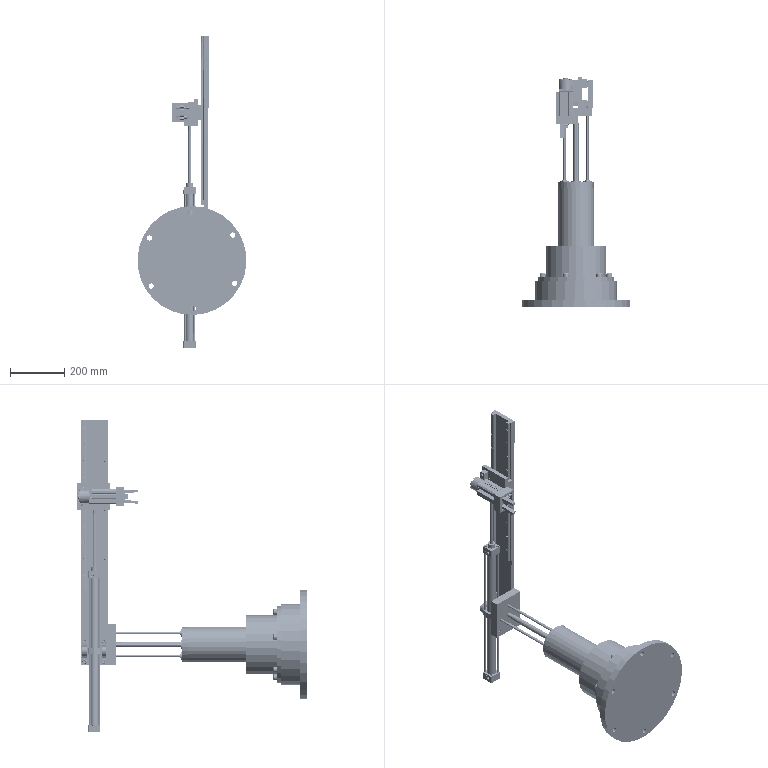Assembly | SolidWorks | mm | 112 component files | 120 solids | 7474 faces | box 400 x 843.52 x 1146.48 mm | volume 16441186 mm3 | plane 3446 | cylinder 1850 | spline 841 | cone 540 | torus 485 | sphere 312 | commonest cylinder face diameters 8 x158 4 x120 14.98 x112 6 x92 15 x81 3 x74 4.8 x68 1 x58
Bill of materials:
15LinearRailSlider | 2 |  | Tall rectangular block with a full-length slot cut into one face; the slot has a profile with small semicircular reliefs at its inner corners. Also has a stepped, counterbored hole on the top face, cross holes on a side face, and a thin raised strip along one side.
15x620LinearRail | 2 |  | Long, slender straight bar with a constant cross-section and a row of evenly spaced small holes along its length. The end profile is roughly I- or hourglass-shaped, with concave cutouts and angled notches on both long sides.
ArmGrippingGear | 2 |  | Straight-toothed spur-gear-like cylinder with a through bore and a single rectangular keyway notch in the bore.
ArmGrippingRack | 1 |  | Rectangular prismatic block with straight, evenly spaced trapezoidal teeth cut along two opposite faces, like a double-sided rack.
ArmRotationCylinderConnectionBlock | 1 |  | Rectangular block with a square cross-section and four round holes in a line along one face: two larger holes near the ends and two smaller holes near the middle.
ArmTelescopicCylinderPistonRod | 1 |  | Long, thin cylindrical rod with a short reduced-diameter step at one end.
Base | 1 |  | Solid round disc with a flange and a raised cylindrical boss on one side. There are six small holes evenly spaced around the edge of the flange.
BearingOuterMountingSleeve | 1 |  | Flanged cylindrical sleeve or tube: a thin annular flange with six small holes evenly spaced around it, joined to a hollow cylindrical body with a large central bore.
ClampingPlate | 2 |  | Rectangular bar with a single round hole near one end, passing across the bar's thickness.
ColumnCylinderPistonRod | 1 |  | Solid cylindrical pin or shaft with one stepped end of reduced diameter.
ColumnLiftingCylinderBody | 1 |  | Multi-body or assembled-looking shape: two square end blocks with rounded corners are joined by a central cylindrical tube and four slender rods, one near each corner. A short cylindrical protrusion sticks out from one end block.
ColumnRotationCylinderFlangePlate | 1 |  | Flat solid disc with a small central bore that has a single rectangular keyway notch.
ColumnSmallArmConnectionPlate | 1 |  | Flat rectangular plate with one larger central hole and eight smaller holes arranged around it: four near the corners and four near the edge midpoints.
CylindricalUpperFlangePlate | 1 |  | Thick round disc with a large central bore and several rings of holes: four large holes, four small inner holes, and four medium holes near the rim.
FixedPost | 1 |  | Straight hollow cylindrical tube with a constant thin wall and plain square-cut ends.
GrippingMandrel | 2 |  | Solid stepped round shaft: a long small-diameter journal at one end, a larger central body with a narrow raised collar, and a short small-diameter stub at the other end.
GrippingMountingHousing | 1 |  | Rectangular block with a large rectangular cavity open on one face. It has a round through-hole centred in the wall opposite the opening and two small holes on an adjacent side face.
GB_FASTENER_SCREWS_HSHCS M3X10-N | 16 |  | Headed cylindrical pin: a short larger-diameter cylindrical head with a rounded outer edge, and a long plain cylindrical shank with a chamfered end.
GB_FASTENER_SCREWS_HSHCS M14X40-N | 6 |  | Headed cylindrical pin with a cylindrical head with a rounded edge and a plain shank with a chamfered tip; the shank is relatively thicker than in similar parts.
GB_FASTENER_SCREWS_HSHCS M6X20-N | 4 |  | Headed cylindrical pin with a cylindrical head with a rounded edge and a long plain chamfered shank.
GB_FASTENER_SCREWS_HSHCS M8X20-N | 4 |  | Headed cylindrical pin with a stubbier shank: a cylindrical head with a rounded edge and a plain chamfered shank.
GB_FASTENER_SCREWS_HSHCS M8X30-N | 4 |  | Slender headed cylindrical pin with a cylindrical head with a rounded edge and a long plain chamfered shank.
GB_FASTENER_SCREWS_HSHCS M10X25-N | 4 |  | Headed cylindrical pin with a relatively large head and a shorter plain chamfered shank.
GB_FASTENER_SCREWS_HSHCS M4X16-N | 28 |  | Long slender headed cylindrical pin with a short cylindrical head with a rounded edge and a long plain chamfered shank.
GB_FASTENER_SCREWS_HSHCS M6X12-N | 2 |  | Stout headed cylindrical pin with a large cylindrical head with a rounded edge and a thick, relatively short plain chamfered shank.
GB_FASTENER_SCREWS_HSHCS M5X20-N | 1 |  | Headed cylindrical part with a hexagonal socket recess in the head; the form resembles a socket-head cap screw, but no threads are modeled.
LiftingRod | 4 |  | Long, slender, solid cylindrical rod with plain ends.
LinearRailConnectionPlate | 1 |  | L-shaped thin plate or bracket: a long narrow upright strip with a short perpendicular return flange at its lower end. Both faces of the lower corner region have a pattern of four small holes.
RackAndPinionRotaryActuatorCDRA1BS50-180CZ | 1 |  | Compact rectangular prismatic body with a square end face. The end face has four socket-head cap screws at its corners. The body has long grooves along its sides, several round side ports or holes, and a cylindrical shaft sticking out from one side face.
MiddleEarFixingBlock1 | 1 |  | Clevis-style bracket: a flat rectangular mounting bar with rounded corners and two through-holes, plus a tapered tongue sticking out perpendicular from the middle of the bar. The tongue ends in a rounded eye with one through-hole.
MiddleEarFixingBlock2 | 1 |  | Clevis-style bracket: a flat rectangular mounting bar with rounded corners and two through-holes, plus a tapered tongue sticking out perpendicular from the middle of the bar. The tongue ends in a rounded eye with one through-hole.
MiddleEarFixingConnectionBlock | 1 |  | Block with a large central through-bore and four smaller through-holes around it. The outline is an irregular hexagon with rectangular tabs on two opposite sides. Two coaxial cylindrical pins (trunnions) stick out from those opposite sides.
RobotArmTelescopicCylinderBody | 1 |  | Long, slender, square-section column: square end caps at both ends, a central tube, and four thin rods running along the corners between the caps. A small round boss with a central hole sticks out from one end cap.
RoundFlangeLinearBearingD8 | 4 |  | Flanged cylindrical bushing or housing: a thin round flange with four equally spaced through-holes and a cylindrical hub on one side. A central through-bore has concentric ring features at the hub end.
SlideRailCarriage | 1 |  | Flat rectangular plate of uniform thickness with ten through-holes: eight small holes in two rectangular four-hole groups and two larger holes arranged vertically near one end.
Rolling bearings 32026 GB 297-94 | 2 |  | Annular rolling-element bearing-like assembly: an outer ring, an inner ring, and a ring of many rolling elements separated by thin webs, with the inner ring standing out axially on one face.
TelescopicCylinderConnectionBlock | 1 |  | Rectangular block with a single round through-hole running through its thickness.
VaneRotaryActuatorCRBU2S30-180 | 1 |  | Housing with a square flange and a cylindrical body. A stepped output shaft with a flat sticks out from the flange face; the body has side pads with holes.
WristClampingCylinderBody | 1 |  | Extruded square-section body with clipped corners, four corner through-holes, a central bore, lengthwise slots or grooves on the outside, and a slotted tab on one side.
WristClampingPistonRod | 1 |  | Stepped round pin or shaft: a long section of larger diameter and a shorter, smaller-diameter section at one end.
Mates:
1. concentric | Base-1 face at (-87.309, 91.019, 566.392) dir (0, -1, 0) r 150 | FixedPost-1 face at (-87.309, 528.019, 566.392) dir (0, -1, 0) r 55
2. concentric | RoundFlangeLinearBearingD8-2 face at (-88.775, 553.019, 608.366) dir (0, 1, 0) r 7.5 | LiftingRod-2 face at (-88.775, 796.583, 608.366) dir (0, -1, 0) r 4
3. width | RackAndPinionRotaryActuatorCDRA1BS50-180CZ-1 face at (-116.161, 145.519, 504.347) dir (-0.9994, 0, -0.0349) | RackAndPinionRotaryActuatorCDRA1BS50-180CZ-1 face at (-54.199, 145.519, 506.511) dir (0.9994, 0, 0.0349) | Base-1 face at (-130.164, 126.019, 647.446) dir (0.9994, 0, 0.0349) | Base-1 face at (-50.213, 126.019, 650.237) dir (-0.9994, 0, -0.0349)
4. width | RackAndPinionRotaryActuatorCDRA1BS50-180CZ-1 face at (-102.231, 186.394, 487.823) dir (0.0349, 0, -0.9994) | RackAndPinionRotaryActuatorCDRA1BS50-180CZ-1 face at (-107.675, 127.644, 643.728) dir (-0.0349, 0, 0.9994) | Base-1 face at (-124.406, 126.019, 482.546) dir (-0.0349, 0, 0.9994) | Base-1 face at (-130.164, 126.019, 647.446) dir (0.0349, 0, -0.9994)
5. coincident | Base-1 face at (-87.309, 126.019, 566.392) dir (0, 1, 0) | RackAndPinionRotaryActuatorCDRA1BS50-180CZ-1 face at (-98.388, 126.019, 504.968) dir (0, -1, 0)
6. concentric | FixedPost-1 face at (-87.309, 528.019, 566.392) dir (0, -1, 0) r 65 | ColumnRotationCylinderFlangePlate-1 face at (-87.309, 208.019, 566.392) dir (0, -1, 0) r 65
7. coincident | RackAndPinionRotaryActuatorCDRA1BS50-180CZ-1 face at (-98.522, 188.019, 543.628) dir (0, 1, 0) | ColumnRotationCylinderFlangePlate-1 face at (-87.309, 188.019, 566.392) dir (0, -1, 0)
8. coincident | FixedPost-1 face at (-87.309, 208.019, 566.392) dir (0, -1, 0) | ColumnRotationCylinderFlangePlate-1 face at (-87.309, 208.019, 566.392) dir (0, 1, 0)
9. concentric | ColumnLiftingCylinderSC50x200-1/ColumnLiftingCylinderBody-1 face at (-87.309, 500.519, 566.392) dir (0, -1, 0) r 25 | FixedPost-1 face at (-87.309, 528.019, 566.392) dir (0, -1, 0) r 65
10. parallel | ColumnLiftingCylinderSC50x200-1/ColumnLiftingCylinderBody-1 face at (-55.354, 235.019, 539.591) dir (0.9994, 0, 0.0349) | Base-1 face at (-130.164, 126.019, 647.446) dir (0.9994, 0, 0.0349)
11. coincident | assembly face at (-87.309, 585.457, 566.392) dir (0, 1, 0) | LiftingRod-2 face at (-88.775, 796.583, 608.366) dir (0, 1, 0)
12. coincident | assembly face at (-87.309, 585.457, 566.392) dir (0, 1, 0) | LiftingRod-2 face at (-88.775, 796.583, 608.366) dir (0, 1, 0)
13. parallel | RobotArmTelescopicCylinderSC32x500-1/MiddleEarFixingBlock1-1 face at (-42.39, 897.583, 491.343) dir (1, 0, -0.00108) | LinearRailConnectionPlate-1 face at (-41.904, 871.583, 941.343) dir (-1, 0, 0.00108)
14. parallel | ColumnSmallArmConnectionPlate-1 face at (-27.228, 806.583, 641.327) dir (1, 0, -0.00108) | LinearRailConnectionPlate-1 face at (-41.904, 871.583, 941.343) dir (-1, 0, 0.00108)
15. coincident | RobotArmTelescopicCylinderSC32x500-1/MiddleEarFixingBlock1-1 face at (-42.39, 897.583, 491.343) dir (1, 0, -0.00108) | LinearRailConnectionPlate-1 face at (-41.904, 871.583, 941.343) dir (-1, 0, 0.00108)
16. width | RobotArmTelescopicCylinderSC32x500-1/MiddleEarFixingBlock2-1 face at (-42.282, 826.583, 591.343) dir (0, -1, 0) | RobotArmTelescopicCylinderSC32x500-1/MiddleEarFixingBlock1-1 face at (-42.282, 916.583, 591.343) dir (0, 1, 0) | LinearRailConnectionPlate-1 face at (-41.418, 921.583, 1391.343) dir (0, 1, 0) | LinearRailConnectionPlate-1 face at (-41.418, 821.583, 1391.343) dir (0, -1, 0)
17. concentric | ColumnLiftingCylinderSC50x200-1/ColumnLiftingCylinderBody-1 face at (-87.309, 527.519, 566.392) dir (0, -1, 0) r 19 | CylindricalUpperFlangePlate-3 face at (-87.309, 548.019, 566.392) dir (0, -1, 0) r 19
18. coincident | ColumnLiftingCylinderSC50x200-1/ColumnLiftingCylinderBody-1 face at (-58.452, 528.019, 539.482) dir (0, 1, 0) | CylindricalUpperFlangePlate-3 face at (-87.309, 528.019, 566.392) dir (0, -1, 0)
19. coincident | FixedPost-1 face at (-87.309, 528.019, 566.392) dir (0, 1, 0) | CylindricalUpperFlangePlate-3 face at (-87.309, 528.019, 566.392) dir (0, -1, 0)
20. parallel | Base-1 face at (-130.164, 126.019, 647.446) dir (0.9994, 0, 0.0349) | CylindricalUpperFlangePlate-3 plane at (-87.309, 528.019, 566.392) dir (0.9994, 0, 0.0349)
21. coincident | RoundFlangeLinearBearingD8-2 face at (-88.775, 553.019, 608.366) dir (0, 1, 0) r 7.5 | CylindricalUpperFlangePlate-3 edge at (-88.775, 548.019, 608.366) dir (0, 1, 0) r 7.5
22. coincident | RoundFlangeLinearBearingD8-2 face at (-88.377, 548.019, 592.371) dir (0, -1, 0) | CylindricalUpperFlangePlate-3 face at (-87.309, 548.019, 566.392) dir (0, 1, 0)
23. width | LinearRailConnectionPlate-1 face at (-42.39, 921.583, 491.343) dir (-0.00108, 0, -1) | LinearRailConnectionPlate-1 face at (-27.228, 821.583, 641.327) dir (0.00108, 0, 1) | ColumnSmallArmConnectionPlate-1 face at (-27.228, 806.583, 641.327) dir (0.00108, 0, 1) | ColumnSmallArmConnectionPlate-1 face at (-27.39, 806.583, 491.327) dir (-0.00108, 0, -1)
24. concentric | assembly face at (-87.309, 585.457, 566.392) dir (0, -1, 0) r 8 | ColumnSmallArmConnectionPlate-1 sketch segment at (-87.309, 806.583, 566.392) dir (0, 1, 0) r 19
25. coincident | ColumnSmallArmConnectionPlate-1 face at (-27.228, 806.583, 641.327) dir (1, 0, -0.00108) | LinearRailConnectionPlate-1 face at (-26.904, 871.583, 941.327) dir (1, 0, -0.00108)
26. coincident | ColumnSmallArmConnectionPlate-1 face at (-87.309, 806.583, 566.392) dir (0, 1, 0) | LinearRailConnectionPlate-1 face at (-27.39, 806.583, 491.327) dir (0, -1, 0)
27. parallel | Base-1 face at (-50.213, 126.019, 650.237) dir (-0.9994, 0, -0.0349) | CylindricalUpperFlangePlate-3 plane at (-87.309, 528.019, 566.392) dir (0.9994, 0, 0.0349)
28. concentric | RoundFlangeLinearBearingD8-2 edge at (-100.771, 549.719, 608.068) dir (0, -1, 0) r 1.7 | CylindricalUpperFlangePlate-3 edge at (-100.771, 548.019, 608.068) dir (0, 1, 0) r 1.5
29. concentric | RoundFlangeLinearBearingD8-2 face at (-89.073, 548.019, 620.362) dir (0, -1, 0) r 3.25 | hexagon socket head cap screws gb-1 face at (-89.073, 539.719, 620.362) dir (0, 1, 0) r 1.5
30. coincident | RoundFlangeLinearBearingD8-2 face at (-89.154, 549.719, 623.611) dir (0, 1, 0) | hexagon socket head cap screws gb-1 face at (-89.073, 549.719, 620.362) dir (0, -1, 0)
31. concentric | CylindricalUpperFlangePlate-3 edge at (-109.975, 541.219, 542.086) dir (0, 1, 0) r 3.3 | hexagon socket head cap screws gb-17 edge at (-109.975, 541.219, 542.086) dir (0, -1, 0) r 3
32. coincident | CylindricalUpperFlangePlate-3 face at (-106.677, 541.219, 542.201) dir (0, 1, 0) | hexagon socket head cap screws gb-17 face at (-109.975, 541.219, 542.086) dir (0, -1, 0)
33. concentric | LinearRailConnectionPlate-1 face at (-132.363, 821.583, 516.44) dir (0, 1, 0) r 7.5 | hexagon socket head cap screws gb-21 face at (-132.363, 792.583, 516.44) dir (0, 1, 0) r 4
34. coincident | LinearRailConnectionPlate-1 face at (-136.863, 812.583, 516.445) dir (0, 1, 0) | hexagon socket head cap screws gb-21 face at (-132.363, 812.583, 516.44) dir (0, -1, 0)
35. concentric | CylindricalUpperFlangePlate-3 face at (-131.19, 548.019, 607.312) dir (0, 1, 0) r 4.25 | hexagon socket head cap screws gb-25 face at (-131.19, 518.019, 607.312) dir (0, 1, 0) r 4
36. coincident | CylindricalUpperFlangePlate-3 face at (-87.309, 548.019, 566.392) dir (0, 1, 0) | hexagon socket head cap screws gb-25 face at (-131.19, 548.019, 607.312) dir (0, -1, 0)
37. concentric | FixedPost-1 face at (-87.309, 528.019, 566.392) dir (0, -1, 0) r 65 | tapered roller bearings gb-10 face at (-87.309, 306.019, 566.392) dir (0, 1, 0) r 65
38. concentric | FixedPost-1 face at (-87.309, 528.019, 566.392) dir (0, -1, 0) r 65 | tapered roller bearings gb-9 face at (-87.309, 208.019, 566.392) dir (0, -1, 0) r 65
39. concentric | Base-1 face at (-87.309, 91.019, 566.392) dir (0, -1, 0) r 150 | BearingOuterMountingSleeve-1 face at (-87.309, 186.019, 566.392) dir (0, -1, 0) r 110
40. coincident | Base-1 face at (-87.309, 186.019, 566.392) dir (0, 1, 0) | BearingOuterMountingSleeve-1 face at (-21.667, 186.019, 641.832) dir (0, -1, 0)
41. coincident | FixedPost-1 edge at (-87.309, 208.019, 566.392) dir (0, 1, 0) r 65 | tapered roller bearings gb-9 face at (-87.309, 208.019, 566.392) dir (0, -1, 0)
42. coincident | tapered roller bearings gb-10 face at (-87.309, 306.019, 566.392) dir (0, 1, 0) | BearingOuterMountingSleeve-1 edge at (-87.309, 306.019, 566.392) dir (0, 1, 0) r 65
43. concentric | ColumnSmallArmConnectionPlate-1 face at (-85.843, 791.583, 524.417) dir (0, -1, 0) r 4 | LiftingRod-4 face at (-85.843, 796.583, 524.417) dir (0, -1, 0) r 4
44. concentric | ColumnSmallArmConnectionPlate-1 face at (-129.284, 791.583, 564.926) dir (0, -1, 0) r 4 | LiftingRod-3 face at (-129.284, 796.583, 564.926) dir (0, -1, 0) r 4
45. concentric | ColumnSmallArmConnectionPlate-1 face at (-88.775, 791.583, 608.366) dir (0, -1, 0) r 4 | LiftingRod-2 face at (-88.775, 796.583, 608.366) dir (0, -1, 0) r 4
46. coincident | RobotArmTelescopicCylinderSC32x500-1/MiddleEarFixingBlock1-1 face at (-53.39, 897.583, 491.355) dir (-0.00108, 0, -1) | LinearRailConnectionPlate-1 face at (-42.39, 921.583, 491.343) dir (-0.00108, 0, -1)
47. coincident | LinearRailConnectionPlate-1 face at (-41.904, 871.583, 941.343) dir (-1, 0, 0.00108) | 15x620LinearRail-1 face at (-41.418, 904.112, 1391.343) dir (1, 0, -0.00108)
48. parallel | LinearRailConnectionPlate-1 face at (-41.418, 921.583, 1391.343) dir (0, 1, 0) | 15x620LinearRail-1 face at (-48.317, 916.583, 1391.35) dir (0, 1, 0)
49. coincident | LinearRailConnectionPlate-1 face at (-41.418, 921.583, 1391.343) dir (0.00108, 0, 1) | 15x620LinearRail-1 face at (-43.31, 918.112, 1391.345) dir (0.00108, 0, 1)
50. distance | 15x620LinearRail-1 face at (-48.317, 916.583, 1391.35) dir (0, 1, 0) | LinearRailConnectionPlate-1 face at (-41.418, 921.583, 1391.343) dir (0, 1, 0)
51. width | 15LinearRailSlider-1 face at (-46.073, 916.792, 1081.267) dir (0, -1, 0) | 15LinearRailSlider-1 face at (-48.605, 905.432, 1081.27) dir (0, 1, 0) | 15x620LinearRail-1 face at (-52.248, 918.612, 1391.354) dir (0, 1, 0) | 15x620LinearRail-1 face at (-52.248, 903.612, 1391.354) dir (0, -1, 0)
52. coincident | 15x620LinearRail-1 face at (-53.918, 916.942, 1391.356) dir (-1, 0, 0.00108) | 15LinearRailSlider-1 face at (-54.253, 916.942, 1081.276) dir (1, 0, -0.00108)
53. concentric | RobotArmTelescopicCylinderSC32x500-1/MiddleEarFixingBlock1-1 edge at (-53.377, 907.083, 503.855) dir (1, 0, -0.00108) r 6 | hexagon socket head cap screws gb-29 edge at (-53.377, 907.083, 503.855) dir (1, 0, -0.00108) r 5
54. coincident | RobotArmTelescopicCylinderSC32x500-1/MiddleEarFixingBlock1-1 face at (-53.282, 897.583, 591.355) dir (-1, 0, 0.00108) | hexagon socket head cap screws gb-29 face at (-53.377, 907.083, 503.855) dir (1, 0, -0.00108)
55. concentric | 15x620LinearRail-1 face at (-54.534, 911.112, 821.356) dir (-1, 0, 0.00108) r 4 | hexagon socket head cap screws gb-34 face at (-33.934, 911.112, 821.334) dir (-1, 0, 0.00108) r 2
56. coincident | 15x620LinearRail-1 face at (-49.934, 913.512, 821.352) dir (-1, 0, 0.00108) | hexagon socket head cap screws gb-34 face at (-49.934, 911.112, 821.352) dir (1, 0, -0.00108)
57. concentric | 15x620LinearRail-3 face at (-53.95, 832.054, 1361.356) dir (-1, 0, 0.00108) r 4 | hexagon socket head cap screws gb-64 face at (-33.35, 832.054, 1361.334) dir (-1, 0, 0.00108) r 2
58. coincident | 15x620LinearRail-3 edge at (-49.35, 832.054, 1361.351) dir (-1, 0, 0.00108) r 4 | hexagon socket head cap screws gb-64 face at (-49.35, 832.054, 1361.351) dir (1, 0, -0.00108)
59. coincident | SlideRailCarriage-1 face at (-65.542, 874.54, 1109.688) dir (1, 0, -0.00108) | 15LinearRailSlider-1 face at (-65.395, 866.112, 1245.688) dir (-1, 0, 0.00108)
60. width | SlideRailCarriage-1 face at (-65.488, 934.54, 1159.688) dir (0.00108, 0, 1) | SlideRailCarriage-1 face at (-65.596, 934.54, 1059.688) dir (-0.00108, 0, -1) | 15LinearRailSlider-1 face at (-43.512, 866.112, 1138.065) dir (0.00108, 0, 1) | 15LinearRailSlider-1 face at (-43.573, 866.112, 1081.265) dir (-0.00108, 0, -1)
61. coincident | SlideRailCarriage-1 face at (-80.542, 874.54, 1109.705) dir (-1, 0, 0.00108) | ArmRotationCylinderConnectionBlock-1 face at (-80.499, 924.54, 1149.704) dir (1, 0, -0.00108)
62. concentric | SlideRailCarriage-1 face at (-80.556, 845.054, 1096.705) dir (-1, 0, 0.00108) r 2.25 | hexagon socket head cap screws gb-75 face at (-59.956, 845.054, 1096.682) dir (-1, 0, 0.00108) r 2
63. coincident | SlideRailCarriage-1 face at (-75.956, 842.804, 1096.7) dir (-1, 0, 0.00108) | hexagon socket head cap screws gb-75 face at (-75.956, 845.054, 1096.7) dir (1, 0, -0.00108)
64. concentric | SlideRailCarriage-1 face at (-80.528, 845.054, 1122.705) dir (-1, 0, 0.00108) r 2.25 | hexagon socket head cap screws gb-76 face at (-59.928, 845.054, 1122.682) dir (-1, 0, 0.00108) r 2
65. coincident | SlideRailCarriage-1 face at (-75.928, 842.804, 1122.7) dir (-1, 0, 0.00108) | hexagon socket head cap screws gb-76 face at (-75.928, 845.054, 1122.7) dir (1, 0, -0.00108)
66. concentric | SlideRailCarriage-1 face at (-80.556, 819.054, 1096.705) dir (-1, 0, 0.00108) r 2.25 | hexagon socket head cap screws gb-77 face at (-59.956, 819.054, 1096.682) dir (-1, 0, 0.00108) r 2
67. coincident | SlideRailCarriage-1 face at (-75.956, 816.804, 1096.7) dir (-1, 0, 0.00108) | hexagon socket head cap screws gb-77 face at (-75.956, 819.054, 1096.7) dir (1, 0, -0.00108)
68. concentric | SlideRailCarriage-1 face at (-80.528, 819.054, 1122.705) dir (-1, 0, 0.00108) r 2.25 | hexagon socket head cap screws gb-78 face at (-59.928, 819.054, 1122.682) dir (-1, 0, 0.00108) r 2
69. coincident | SlideRailCarriage-1 face at (-75.928, 816.804, 1122.7) dir (-1, 0, 0.00108) | hexagon socket head cap screws gb-78 face at (-75.928, 819.054, 1122.7) dir (1, 0, -0.00108)
70. concentric | SlideRailCarriage-1 face at (-80.528, 924.112, 1122.705) dir (-1, 0, 0.00108) r 2.25 | hexagon socket head cap screws gb-79 face at (-59.928, 924.112, 1122.682) dir (-1, 0, 0.00108) r 2
71. coincident | SlideRailCarriage-1 face at (-75.928, 921.862, 1122.7) dir (-1, 0, 0.00108) | hexagon socket head cap screws gb-79 face at (-75.928, 924.112, 1122.7) dir (1, 0, -0.00108)
72. concentric | SlideRailCarriage-1 face at (-80.556, 924.112, 1096.705) dir (-1, 0, 0.00108) r 2.25 | hexagon socket head cap screws gb-80 face at (-59.956, 924.112, 1096.682) dir (-1, 0, 0.00108) r 2
73. coincident | SlideRailCarriage-1 face at (-75.956, 921.862, 1096.7) dir (-1, 0, 0.00108) | hexagon socket head cap screws gb-80 face at (-75.956, 924.112, 1096.7) dir (1, 0, -0.00108)
74. concentric | SlideRailCarriage-1 face at (-80.556, 898.112, 1096.705) dir (-1, 0, 0.00108) r 2.25 | hexagon socket head cap screws gb-81 face at (-59.956, 898.112, 1096.682) dir (-1, 0, 0.00108) r 2
75. coincident | SlideRailCarriage-1 face at (-75.956, 895.862, 1096.7) dir (-1, 0, 0.00108) | hexagon socket head cap screws gb-81 face at (-75.956, 898.112, 1096.7) dir (1, 0, -0.00108)
76. concentric | SlideRailCarriage-1 face at (-80.528, 898.112, 1122.705) dir (-1, 0, 0.00108) r 2.25 | hexagon socket head cap screws gb-82 face at (-59.928, 898.112, 1122.682) dir (-1, 0, 0.00108) r 2
77. coincident | SlideRailCarriage-1 face at (-75.928, 895.862, 1122.7) dir (-1, 0, 0.00108) | hexagon socket head cap screws gb-82 face at (-75.928, 898.112, 1122.7) dir (1, 0, -0.00108)
78. width | ArmRotationCylinderConnectionBlock-1 face at (-100.499, 924.54, 1149.726) dir (0.00108, 0, 1) | ArmRotationCylinderConnectionBlock-1 face at (-100.585, 924.54, 1069.726) dir (-0.00108, 0, -1) | SlideRailCarriage-1 face at (-65.596, 934.54, 1059.688) dir (-0.00108, 0, -1) | SlideRailCarriage-1 face at (-65.488, 934.54, 1159.688) dir (0.00108, 0, 1)
79. concentric | SlideRailCarriage-1 face at (-80.575, 914.54, 1079.705) dir (-1, 0, 0.00108) r 3 | ArmRotationCylinderConnectionBlock-1 face at (-100.575, 914.54, 1079.726) dir (-1, 0, 0.00108) r 5.5
80. concentric | VaneRotaryActuatorCRBU2S30-180-1 face at (-110.05, 914.54, 1102.736) dir (1, 0, -0.00108) r 2.5 | ArmRotationCylinderConnectionBlock-1 edge at (-100.55, 914.54, 1102.726) dir (1, 0, -0.00108) r 2.75
81. coincident | VaneRotaryActuatorCRBU2S30-180-1 face at (-100.555, 902.54, 1097.726) dir (1, 0, -0.00108) | ArmRotationCylinderConnectionBlock-1 face at (-100.499, 924.54, 1149.726) dir (-1, 0, 0.00108)
82. concentric | ArmRotationCylinderConnectionBlock-1 face at (-100.51, 914.54, 1139.726) dir (-1, 0, 0.00108) r 3.3 | hexagon socket head cap screws gb-88 face at (-74.51, 914.54, 1139.698) dir (-1, 0, 0.00108) r 3
83. coincident | ArmRotationCylinderConnectionBlock-1 face at (-86.51, 917.84, 1139.711) dir (-1, 0, 0.00108) | hexagon socket head cap screws gb-88 face at (-86.51, 914.54, 1139.711) dir (1, 0, -0.00108)
84. concentric | ArmRotationCylinderConnectionBlock-1 face at (-100.575, 914.54, 1079.726) dir (-1, 0, 0.00108) r 3.3 | hexagon socket head cap screws gb-89 face at (-74.575, 914.54, 1079.698) dir (-1, 0, 0.00108) r 3
85. coincident | ArmRotationCylinderConnectionBlock-1 face at (-86.575, 917.84, 1079.711) dir (-1, 0, 0.00108) | hexagon socket head cap screws gb-89 face at (-86.575, 914.54, 1079.711) dir (1, 0, -0.00108)
86. concentric | ArmRotationCylinderConnectionBlock-1 face at (-80.535, 914.54, 1116.705) dir (1, 0, -0.00108) r 2.75 | hexagon socket head cap screws gb-94 face at (-106.235, 914.54, 1116.732) dir (1, 0, -0.00108) r 2.5
87. coincident | ArmRotationCylinderConnectionBlock-1 face at (-86.235, 917.29, 1116.711) dir (1, 0, -0.00108) | hexagon socket head cap screws gb-94 face at (-86.235, 914.54, 1116.711) dir (-1, 0, 0.00108)
88. coincident | SlideRailCarriage-1 face at (-80.542, 874.54, 1109.705) dir (-1, 0, 0.00108) | TelescopicCylinderConnectionBlock-1 face at (-80.58, 904.54, 1074.705) dir (1, 0, -0.00108)
89. coincident | ArmRotationCylinderConnectionBlock-1 face at (-90.542, 904.54, 1109.715) dir (0, -1, 0) | TelescopicCylinderConnectionBlock-1 face at (-98.088, 904.54, 1067.223) dir (0, 1, 0)
90. coincident | SlideRailCarriage-1 face at (-65.596, 934.54, 1059.688) dir (-0.00108, 0, -1) | TelescopicCylinderConnectionBlock-1 face at (-115.596, 904.54, 1059.742) dir (-0.00108, 0, -1)
91. concentric | RobotArmTelescopicCylinderSC32x500-1/RobotArmTelescopicCylinderBody-1 face at (-96.627, 871.583, 272.402) dir (0.00108, 0, 1) r 6 | ArmTelescopicCylinderPistonRod-1 face at (-95.792, 871.583, 1044.721) dir (-0.00108, 0, -1) r 6
92. distance | ArmTelescopicCylinderPistonRod-1 face at (-95.771, 871.583, 1064.721) dir (0.00108, 0, 1) | TelescopicCylinderConnectionBlock-1 face at (-115.58, 904.54, 1074.742) dir (0.00108, 0, 1)
93. concentric | CylindricalUpperFlangePlate-3 face at (-87.309, 548.019, 566.392) dir (0, -1, 0) r 19 | ColumnCylinderPistonRod-1 face at (-87.309, 766.583, 566.392) dir (0, -1, 0) r 10
94. coincident | LiftingRod-3 face at (-129.284, 796.583, 564.926) dir (0, 1, 0) | ColumnCylinderPistonRod-1 face at (-87.309, 796.583, 566.392) dir (0, 1, 0)
95. distance | ColumnCylinderPistonRod-1 face at (-87.309, 796.583, 566.392) dir (0, 1, 0) | LinearRailConnectionPlate-1 face at (-27.39, 821.583, 491.327) dir (0, 1, 0)
96. coincident | WristClampingAirCTACQS40x50-1/WristClampingCylinderBody-1 face at (-146.265, 881.04, 1088.576) dir (0, 1, 0) | VaneRotaryActuatorCRBU2S30-180-1 face at (-125.542, 881.04, 1109.753) dir (0, -1, 0)
97. parallel | WristClampingAirCTACQS40x50-1/WristClampingCylinderBody-1 face at (-162.049, 899.632, 1103.469) dir (-1, 0, 0.00108) | SlideRailCarriage-1 face at (-80.542, 874.54, 1109.705) dir (-1, 0, 0.00108)
98. concentric | VaneRotaryActuatorCRBU2S30-180-1 face at (-110.035, 914.54, 1116.736) dir (1, 0, -0.00108) r 2.5 | hexagon socket head cap screws gb-94 face at (-106.235, 914.54, 1116.732) dir (1, 0, -0.00108) r 2.5
99. width | WristClampingAirCTACQS40x50-1/WristClampingCylinderBody-1 face at (-146.271, 881.04, 1083.276) dir (-0.00108, 0, -1) | WristClampingAirCTACQS40x50-1/WristClampingCylinderBody-1 face at (-146.213, 881.04, 1136.275) dir (0.00108, 0, 1) | VaneRotaryActuatorCRBU2S30-180-1 face at (-115.895, 890.04, 1135.743) dir (0.00108, 0, 1) | VaneRotaryActuatorCRBU2S30-180-1 face at (-135.189, 890.04, 1083.764) dir (-0.00108, 0, -1)
100. coincident | WristClampingAirCTACQS40x50-1/WristClampingCylinderBody-1 face at (-151.519, 881.04, 1130.981) dir (-1, 0, 0.00108) | VaneRotaryActuatorCRBU2S30-180-1 face at (-151.553, 890.04, 1100.162) dir (-1, 0, 0.00108)
101. concentric | WristClampingAirCTACQS40x50-1/WristClampingCylinderBody-1 face at (-125.042, 874.04, 1109.753) dir (0, -1, 0) r 8 | WristClampingPistonRod-2 face at (-125.042, 776.966, 1109.753) dir (0, 1, 0) r 6
102. concentric | TelescopicCylinderConnectionBlock-1 face at (-95.76, 871.583, 1074.721) dir (0.00108, 0, 1) r 5 | ArmTelescopicCylinderPistonRod-1 face at (-95.771, 871.583, 1064.721) dir (-0.00108, 0, -1) r 5
103. parallel | SlideRailCarriage-1 face at (-80.542, 874.54, 1109.705) dir (-1, 0, 0.00108) | ArmGrippingRack-1 face at (-132.552, 775.395, 1100.736) dir (-1, 0, 0.00108)
104. parallel | SlideRailCarriage-1 face at (-80.542, 874.54, 1109.705) dir (-1, 0, 0.00108) | ArmGrippingGear-1 face at (-117.551, 768.611, 1101.127) dir (1, 0, -0.00108)
105. concentric | WristClampingPistonRod-2 face at (-125.042, 756.966, 1109.753) dir (0, 1, 0) r 4 | ArmGrippingRack-1 face at (-125.042, 756.966, 1109.753) dir (0, 1, 0) r 5
106. coincident | WristClampingPistonRod-2 face at (-125.042, 776.966, 1109.753) dir (0, -1, 0) | ArmGrippingRack-1 face at (-117.531, 776.966, 1119.769) dir (0, 1, 0)
107. rack pinion | ArmGrippingRack-1 sketch segment at (-125.052, 775.395, 1100.728) dir (0, -1, 0) | ArmGrippingGear-1 sketch segment at (-125.061, 765.309, 1092.228) dir (-1, 0, 0.00108) r 8.5
108. coincident | ArmGrippingRack-1 face at (-132.552, 775.395, 1100.736) dir (-1, 0, 0.00108) | ArmGrippingGear-1 face at (-132.561, 765.309, 1092.236) dir (-1, 0, 0.00108)
109. distance | ArmGrippingGear-1 sketch point at (-125.061, 765.309, 1092.228) dir (1, 0, 0) | ArmGrippingRack-1 sketch segment at (-125.052, 775.395, 1100.728) dir (0, -1, 0)
110. concentric | ArmGrippingGear-1 face at (-125.061, 765.309, 1092.228) dir (-1, 0, 0.00108) r 5 | GrippingMandrel-1 face at (-114.642, 765.309, 1092.216) dir (1, 0, -0.00108) r 5
111. concentric | GrippingMandrel-1 face at (-147.642, 765.309, 1092.252) dir (1, 0, -0.00108) r 3 | ClampingPlate-1 face at (-127.642, 765.309, 1092.23) dir (-1, 0, 0.00108) r 3
112. lock | ArmGrippingGear-1 reference at (0, 0, 0) dir (1, 0, 0) | ClampingPlate-1 reference at (0, 0, 0) dir (1, 0, 0)
113. lock | ArmGrippingGear-2 reference at (0, 0, 0) dir (1, 0, 0) | ClampingPlate-3 reference at (0, 0, 0) dir (1, 0, 0)
114. coincident | GrippingMandrel-1 face at (-147.642, 765.309, 1092.252) dir (-1, 0, 0.00108) | ClampingPlate-1 face at (-147.643, 740.362, 1090.631) dir (-1, 0, 0.00108)
115. coincident | GrippingMandrel-1 face at (-147.642, 765.309, 1092.252) dir (-1, 0, 0.00108) | ClampingPlate-1 face at (-147.643, 740.362, 1090.631) dir (-1, 0, 0.00108)
116. coincident | WristClampingAirCTACQS40x50-1/WristClampingCylinderBody-1 face at (-146.265, 791.54, 1088.576) dir (0, -1, 0) | GrippingMountingHousing-2 face at (-92.004, 791.54, 1144.717) dir (0, 1, 0)
117. width | GrippingMountingHousing-2 face at (-92.004, 791.54, 1144.717) dir (0.00108, 0, 1) | GrippingMountingHousing-2 face at (-92.08, 791.54, 1074.717) dir (-0.00108, 0, -1) | WristClampingAirCTACQS40x50-1/WristClampingCylinderBody-1 face at (-146.271, 881.04, 1083.276) dir (-0.00108, 0, -1) | WristClampingAirCTACQS40x50-1/WristClampingCylinderBody-1 face at (-146.213, 881.04, 1136.275) dir (0.00108, 0, 1)
118. coincident | WristClampingAirCTACQS40x50-1/WristClampingCylinderBody-1 face at (-162.049, 899.632, 1103.469) dir (-1, 0, 0.00108) | GrippingMountingHousing-2 face at (-162.042, 776.54, 1109.793) dir (-1, 0, 0.00108)
119. concentric | BearingOuterMountingSleeve-1 face at (-209.195, 201.019, 594.437) dir (0, 1, 0) r 7.75 | hexagon socket head cap screws gb-97 face at (-209.195, 160.019, 594.437) dir (0, 1, 0) r 7
120. coincident | BearingOuterMountingSleeve-1 face at (-215.042, 200.019, 599.524) dir (0, 1, 0) | hexagon socket head cap screws gb-97 face at (-209.195, 200.019, 594.437) dir (0, -1, 0)
121. width | 15LinearRailSlider-3 face at (-46.012, 826.374, 1138.067) dir (0, 1, 0) | 15LinearRailSlider-3 face at (-48.543, 837.734, 1138.07) dir (0, -1, 0) | 15x620LinearRail-3 face at (-52.248, 839.554, 1391.354) dir (0, 1, 0) | 15x620LinearRail-3 face at (-52.248, 824.554, 1391.354) dir (0, -1, 0)
122. coincident | 15x620LinearRail-3 face at (-53.918, 837.884, 1391.356) dir (-1, 0, 0.00108) | 15LinearRailSlider-3 face at (-54.191, 826.223, 1138.076) dir (1, 0, -0.00108)